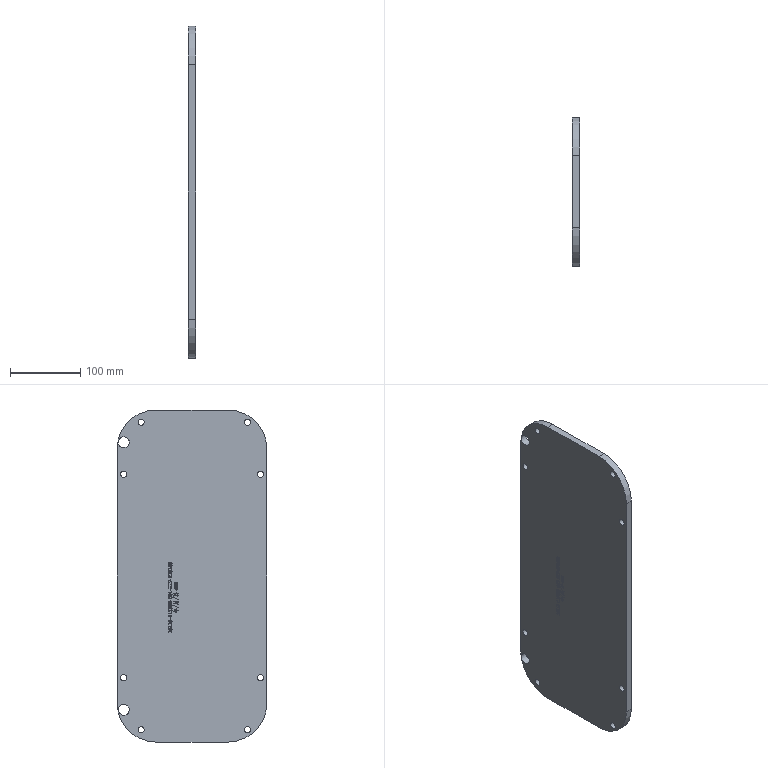CAM job | NX | mm | 3-axis | 4 set-ups | 33 operations | part box 10 x 213 x 473
set-up 1
1. Planar Milling | Mill Mill5 LX-D12 | PLANAR_MILLING_1 | path 8901.97 mm | 2.143 min
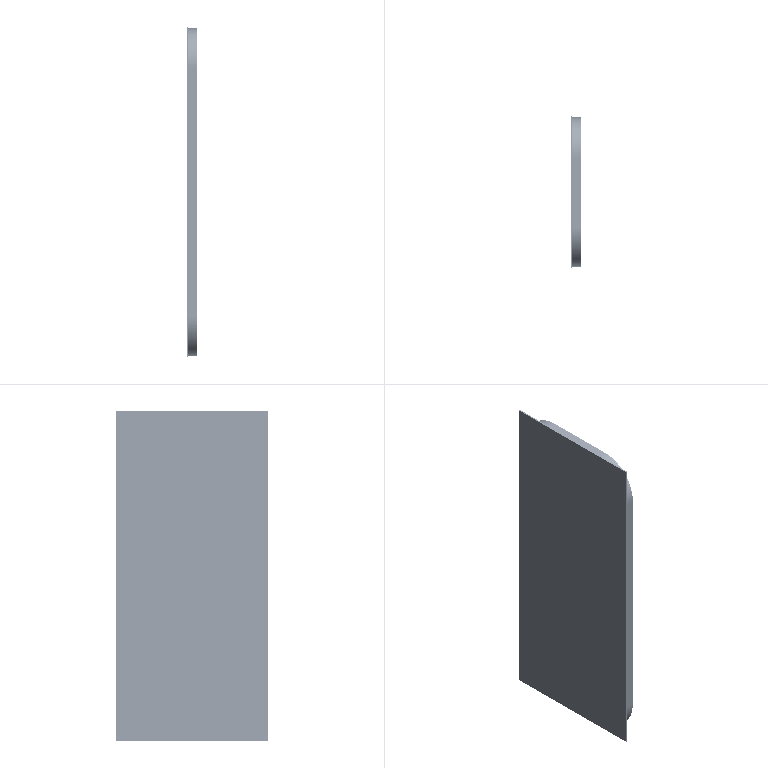2. Planar Milling | Mill Mill5 LX-D12J | PLANAR_MILLING_2 | path 12097.965 mm | 6.053 min
set-up 2
3. Face Milling | Mill Mill5 E50R0.8 | FACE_MILLING_3 | path 8508.5 mm | 2.678 min
set-up 3
4. Face Milling | Mill Mill5 E50R0.8 | FACE_MILLING_4 | path 8504.9 mm | 2.677 min
5. Face Milling | Mill Mill5 E50R0.8 | FACE_MILLING_5 | path 5008.4 mm | 6.22 min
6. Planar Milling | Mill Mill5 LX-D12 | PLANAR_MILLING_6 | path 5352.088 mm | 1.329 min
7. Cylinder Milling | Mill Mill5 LX-D6 | CYLINDER_MILLING_7 | path 2909.311 mm | 2.164 min
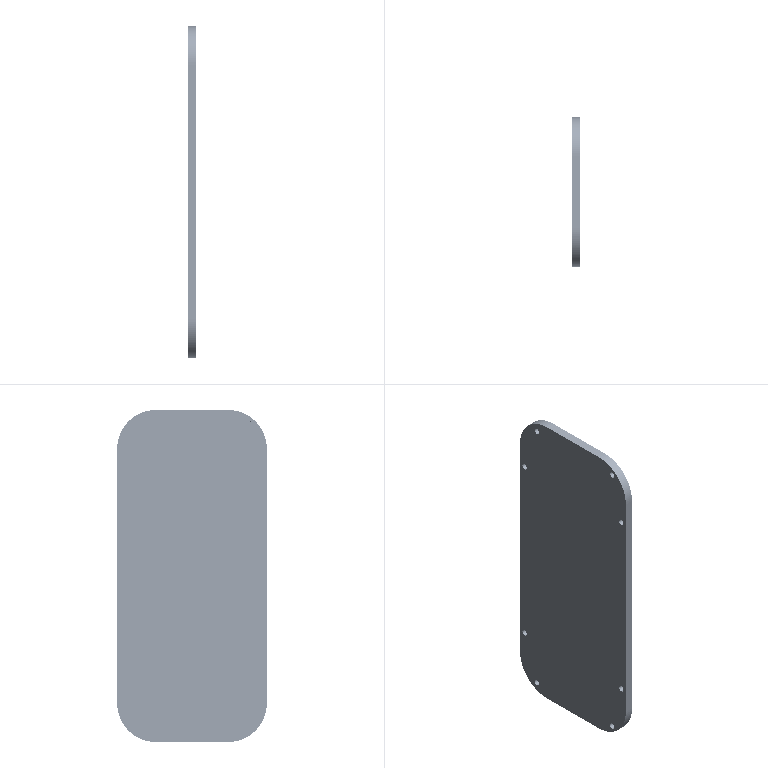8. Cylinder Milling | Mill Mill5 LX-D6J | CYLINDER_MILLING_8 | path 1859.542 mm | 1.577 min
9. Cylinder Milling | Mill Mill5 LX-D10 | CYLINDER_MILLING_9 | path 1090.693 mm | 0.8219 min
10. Cylinder Milling | Mill Mill5 LX-D10J | CYLINDER_MILLING_10 | path 737.73 mm | 0.7038 min
11. Fixed-axis Surface Contouring | Mill MillChamfer DJ-D10A90 | FIXED-AXIS_SURFACE_CONTOURING_11 | path 3315.283 mm | 1.79 min
12. Planar Text | Mill Mill5 KZ-D0.5R0.25 | PLANAR_TEXT_12 | path 2107.016 mm | 1.036 min
13. Planar Text | Mill Mill5 KZ-D0.5R0.25 | PLANAR_TEXT_13 | path 929.841 mm | 0.4787 min
14. Planar Milling | Mill Mill5 LX-D12J | PLANAR_MILLING_14 | path 1394.209 mm | 1.685 min
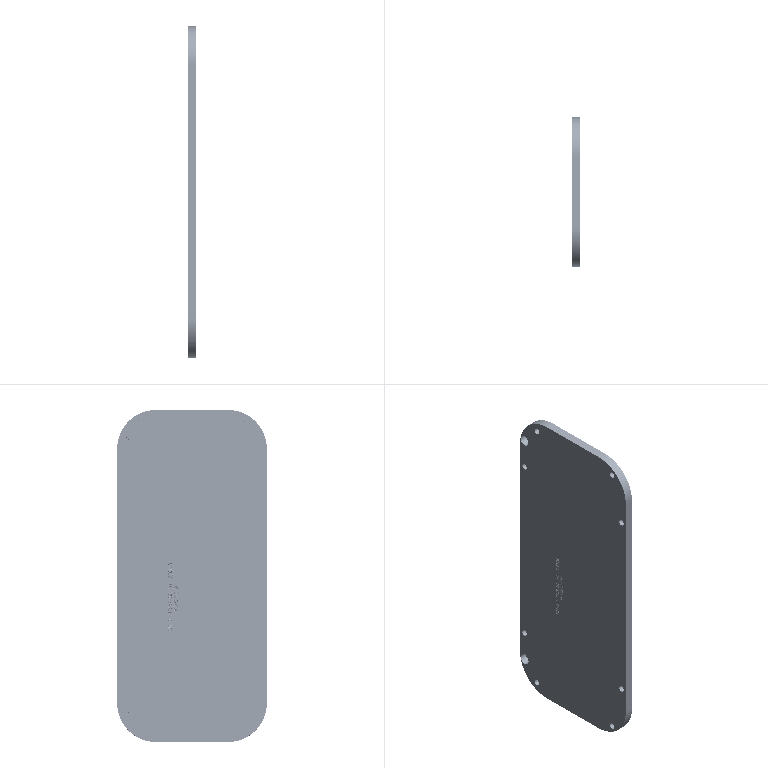15. Planar Milling | Mill Mill5 LX-D12J | PLANAR_MILLING_15 | path 12095.935 mm | 6.053 min
set-up 4
16. Face Milling | Mill Mill5 E50R0.8 | FACE_MILLING_16 | path 8504.9 mm | 2.677 min
17. Cavity Milling | Mill Mill5 LX-D3 | CAVITY_MILLING_17 | path 26869.705 mm | 9.243 min
18. Cavity Milling | Mill Mill5 LX-D2 | CAVITY_MILLING_18 | path 28644.835 mm | 9.9 min
19. Face Milling | Mill Mill5 E50R0.8 | FACE_MILLING_19 | path 5017.4 mm | 6.221 min
20. Cylinder Milling | Mill Mill5 LX-D6 | CYLINDER_MILLING_20 | path 86.996 mm | 0.06159 min
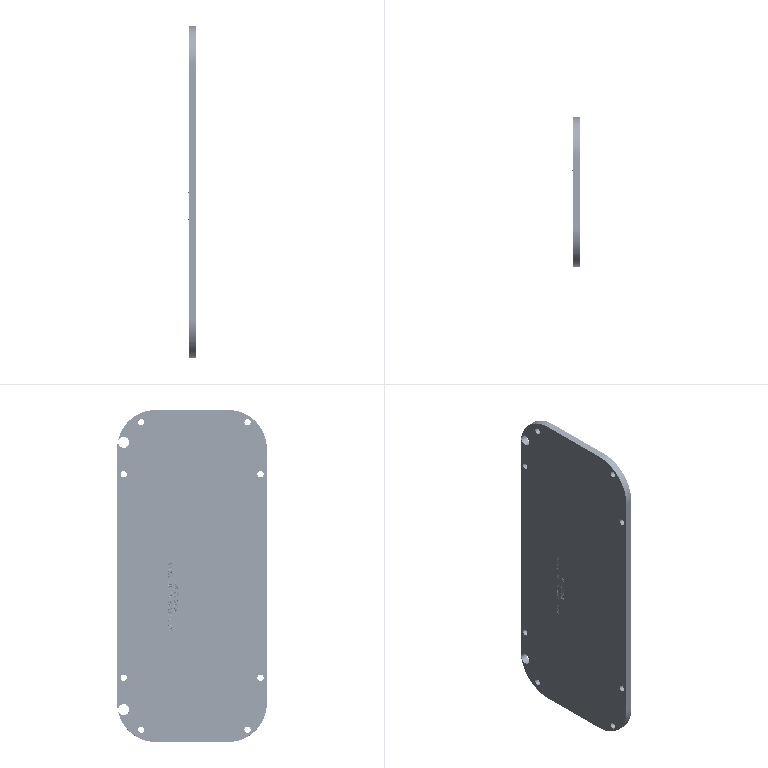21. Cylinder Milling | Mill Mill5 LX-D6J | CYLINDER_MILLING_21 | path 67.658 mm | 0.07094 min
22. Cylinder Milling | Mill Mill5 LX-D4 | CYLINDER_MILLING_22 | path 57.784 mm | 0.02519 min
23. Cylinder Milling | Mill Mill5 LX-D4J | CYLINDER_MILLING_23 | path 58.582 mm | 0.04861 min
24. Volume Based 2.5D Milling | Mill Mill5 LX-D3J | VOLUME_BASED_2.5D_MILLING_24 | path 2200.528 mm | 2.704 min
25. Volume Based 2.5D Milling | Mill Mill5 LX-D2 | VOLUME_BASED_2.5D_MILLING_25 | path 1663.537 mm | 2.033 min
26. Z-Level Milling | Mill Mill5 YB-D3R0.2 | Z-LEVEL_MILLING_26 | path 21450.575 mm | 8.552 min
27. Z-Level Milling | Mill Mill5 YB-D2R0.2 | Z-LEVEL_MILLING_27 | path 8077.262 mm | 3.212 min
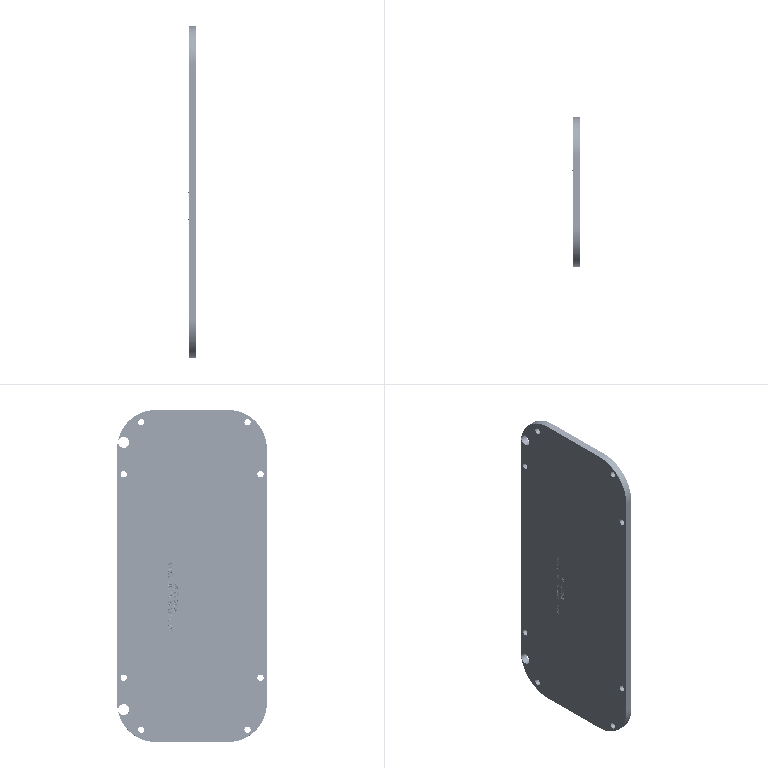28. Planar Milling | Mill Mill5 YW-D7.36A48R0.76 | PLANAR_MILLING_28 | path 1119.575 mm | 3.608 min
29. Planar Milling | Mill Mill5 YW-D7.36A48R0.76 | PLANAR_MILLING_29 | path 1120.225 mm | 3.61 min
30. Planar Milling | Mill Mill5 YW-D4.16A48R0.76 | PLANAR_MILLING_30 | path 846.488 mm | 2.702 min
31. Planar Milling | Mill Mill5 YW-D4.16A48R0.76 | PLANAR_MILLING_31 | path 848.274 mm | 2.708 min
32. Fixed-axis Surface Contouring | Mill MillChamfer DJ-D6A90 | FIXED-AXIS_SURFACE_CONTOURING_32 | path 4260.916 mm | 1.909 min
33. Planar Milling | Mill Mill5 LX-D12J | PLANAR_MILLING_33 | path 5410.019 mm | 2.696 min